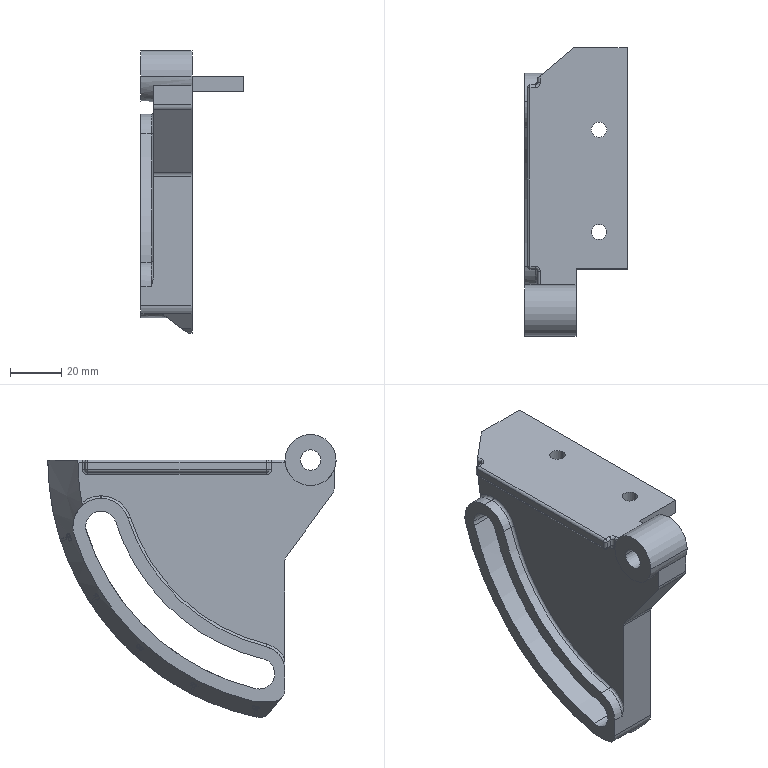Component | SolidWorks | Angle-1 | 1 solid | 300 faces | box 40 x 112.75 x 110.69 mm | volume 76463 mm3 | plane 113 | spline 103 | cylinder 65 | cone 8 | torus 7 | sphere 4 | commonest cylinder face diameters 0.5 x17 2 x15 6 x9 11.98 x5 18 x4 21.98 x3 20 x3 8 x2